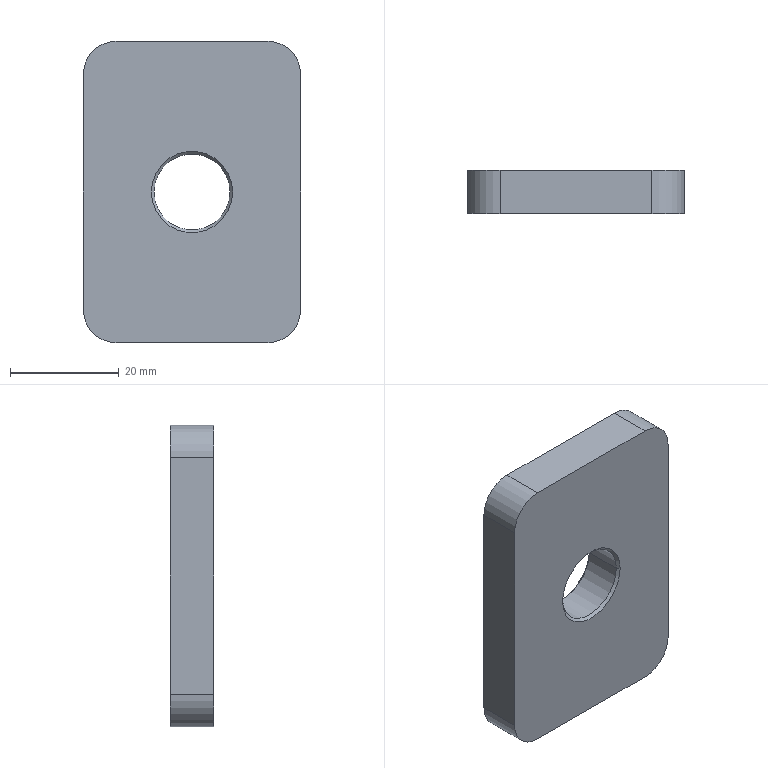Component | SolidWorks | 01-04RearWheelConnectionPlate-4 | 1 solid | 16 faces | box 40 x 8 x 55.5 mm | volume 16270 mm3 | cylinder 6 | plane 6 | cone 4 | commonest cylinder face diameters 12 x4 14 x2 | material Q235
STEP:
#1=CARTESIAN_POINT('',(-12.087,-0.01969,-13.848));
#2=VERTEX_POINT('',#1);
#3=CARTESIAN_POINT('',(-11.535,-0.01969,-13.848));
#4=VERTEX_POINT('',#3);
#5=CARTESIAN_POINT('',(-11.811,-0.01969,-13.848));
#6=DIRECTION('',(-0.,1.,-0.));
#7=DIRECTION('',(-1.,0.,0.));
#8=AXIS2_PLACEMENT_3D('',#5,#6,#7);
#9=CIRCLE('',#8,0.2756);
#10=EDGE_CURVE('',#2,#4,#9,.T.);
#11=ORIENTED_EDGE('',*,*,#10,.F.);
#12=CARTESIAN_POINT('',(-12.106,-0.,-13.848));
#13=VERTEX_POINT('',#12);
#14=CARTESIAN_POINT('',(-12.087,-0.01969,-13.848));
#15=DIRECTION('',(-0.7071,0.7071,0.));
#16=VECTOR('',#15,39.37);
#17=LINE('',#14,#16);
#18=EDGE_CURVE('',#2,#13,#17,.T.);
#19=ORIENTED_EDGE('',*,*,#18,.T.);
#20=CARTESIAN_POINT('',(-11.516,-0.,-13.848));
#21=VERTEX_POINT('',#20);
#22=CARTESIAN_POINT('',(-11.811,-0.,-13.848));
#23=DIRECTION('',(0.,-1.,0.));
#24=DIRECTION('',(-1.,-0.,0.));
#25=AXIS2_PLACEMENT_3D('',#22,#23,#24);
#26=CIRCLE('',#25,0.2953);
#27=EDGE_CURVE('',#21,#13,#26,.T.);
#28=ORIENTED_EDGE('',*,*,#27,.F.);
#29=CARTESIAN_POINT('',(-11.535,-0.01969,-13.848));
#30=DIRECTION('',(0.7071,0.7071,-0.));
#31=VECTOR('',#30,39.37);
#32=LINE('',#29,#31);
#33=EDGE_CURVE('',#4,#21,#32,.T.);
#34=ORIENTED_EDGE('',*,*,#33,.F.);
#35=EDGE_LOOP('',(#11,#19,#28,#34));
#36=FACE_OUTER_BOUND('',#35,.T.);
#37=CARTESIAN_POINT('',(-11.811,-0.01969,-13.848));
#38=DIRECTION('',(-0.,1.,-0.));
#39=DIRECTION('',(1.,0.,0.));
#40=AXIS2_PLACEMENT_3D('',#37,#38,#39);
#41=CONICAL_SURFACE('',#40,0.2756,0.7854);
#42=ADVANCED_FACE('',(#36),#41,.F.);
#43=CARTESIAN_POINT('',(-11.535,-0.2953,-13.848));
#44=VERTEX_POINT('',#43);
#45=CARTESIAN_POINT('',(-12.087,-0.2953,-13.848));
#46=VERTEX_POINT('',#45);
#47=CARTESIAN_POINT('',(-11.811,-0.2953,-13.848));
#48=DIRECTION('',(0.,-1.,0.));
#49=DIRECTION('',(-1.,0.,0.));
#50=AXIS2_PLACEMENT_3D('',#47,#48,#49);
#51=CIRCLE('',#50,0.2756);
#52=EDGE_CURVE('',#44,#46,#51,.T.);
#53=ORIENTED_EDGE('',*,*,#52,.F.);
#54=CARTESIAN_POINT('',(-11.516,-0.315,-13.848));
#55=VERTEX_POINT('',#54);
#56=CARTESIAN_POINT('',(-11.535,-0.2953,-13.848));
#57=DIRECTION('',(0.7071,-0.7071,-0.));
#58=VECTOR('',#57,39.37);
#59=LINE('',#56,#58);
#60=EDGE_CURVE('',#44,#55,#59,.T.);
#61=ORIENTED_EDGE('',*,*,#60,.T.);
#62=CARTESIAN_POINT('',(-12.106,-0.315,-13.848));
#63=VERTEX_POINT('',#62);
#64=CARTESIAN_POINT('',(-11.811,-0.315,-13.848));
#65=DIRECTION('',(-0.,1.,-0.));
#66=DIRECTION('',(-1.,0.,0.));
#67=AXIS2_PLACEMENT_3D('',#64,#65,#66);
#68=CIRCLE('',#67,0.2953);
#69=EDGE_CURVE('',#63,#55,#68,.T.);
#70=ORIENTED_EDGE('',*,*,#69,.F.);
#71=CARTESIAN_POINT('',(-12.087,-0.2953,-13.848));
#72=DIRECTION('',(-0.7071,-0.7071,0.));
#73=VECTOR('',#72,39.37);
#74=LINE('',#71,#73);
#75=EDGE_CURVE('',#46,#63,#74,.T.);
#76=ORIENTED_EDGE('',*,*,#75,.F.);
#77=EDGE_LOOP('',(#53,#61,#70,#76));
#78=FACE_OUTER_BOUND('',#77,.T.);
#79=CARTESIAN_POINT('',(-11.811,-0.2953,-13.848));
#80=DIRECTION('',(0.,-1.,0.));
#81=DIRECTION('',(-1.,0.,0.));
#82=AXIS2_PLACEMENT_3D('',#79,#80,#81);
#83=CONICAL_SURFACE('',#82,0.2756,0.7854);
#84=ADVANCED_FACE('',(#78),#83,.F.);
#85=ORIENTED_EDGE('',*,*,#52,.T.);
#86=CARTESIAN_POINT('',(-12.087,-0.,-13.848));
#87=DIRECTION('',(-0.,1.,-0.));
#88=VECTOR('',#87,39.37);
#89=LINE('',#86,#88);
#90=EDGE_CURVE('',#46,#2,#89,.T.);
#91=ORIENTED_EDGE('',*,*,#90,.T.);
#92=ORIENTED_EDGE('',*,*,#10,.T.);
#93=CARTESIAN_POINT('',(-11.535,-0.,-13.848));
#94=DIRECTION('',(-0.,1.,-0.));
#95=VECTOR('',#94,39.37);
#96=LINE('',#93,#95);
#97=EDGE_CURVE('',#44,#4,#96,.T.);
#98=ORIENTED_EDGE('',*,*,#97,.F.);
#99=EDGE_LOOP('',(#85,#91,#92,#98));
#100=FACE_OUTER_BOUND('',#99,.T.);
#101=CARTESIAN_POINT('',(-11.811,-0.,-13.848));
#102=DIRECTION('',(-0.,1.,-0.));
#103=DIRECTION('',(1.,0.,0.));
#104=AXIS2_PLACEMENT_3D('',#101,#102,#103);
#105=CYLINDRICAL_SURFACE('',#104,0.2756);
#106=ADVANCED_FACE('',(#100),#105,.F.);
#107=ORIENTED_EDGE('',*,*,#27,.T.);
#108=CARTESIAN_POINT('',(-11.811,-0.,-13.848));
#109=DIRECTION('',(0.,-1.,0.));
#110=DIRECTION('',(-1.,-0.,0.));
#111=AXIS2_PLACEMENT_3D('',#108,#109,#110);
#112=CIRCLE('',#111,0.2953);
#113=EDGE_CURVE('',#13,#21,#112,.T.);
#114=ORIENTED_EDGE('',*,*,#113,.T.);
#115=EDGE_LOOP('',(#107,#114));
#116=FACE_BOUND('',#115,.T.);
#117=CARTESIAN_POINT('',(-11.26,-0.,-14.941));
#118=VERTEX_POINT('',#117);
#119=CARTESIAN_POINT('',(-11.024,-0.,-14.705));
#120=VERTEX_POINT('',#119);
#121=CARTESIAN_POINT('',(-11.26,-0.,-14.705));
#122=DIRECTION('',(0.,-1.,0.));
#123=DIRECTION('',(-1.,-0.,0.));
#124=AXIS2_PLACEMENT_3D('',#121,#122,#123);
#125=CIRCLE('',#124,0.2362);
#126=EDGE_CURVE('',#118,#120,#125,.T.);
#127=ORIENTED_EDGE('',*,*,#126,.F.);
#128=CARTESIAN_POINT('',(-12.362,-0.,-14.941));
#129=VERTEX_POINT('',#128);
#130=CARTESIAN_POINT('',(-12.362,-0.,-14.941));
#131=DIRECTION('',(1.,0.,-0.));
#132=VECTOR('',#131,39.37);
#133=LINE('',#130,#132);
#134=EDGE_CURVE('',#129,#118,#133,.T.);
#135=ORIENTED_EDGE('',*,*,#134,.F.);
#136=CARTESIAN_POINT('',(-12.598,-0.,-14.705));
#137=VERTEX_POINT('',#136);
#138=CARTESIAN_POINT('',(-12.362,-0.,-14.705));
#139=DIRECTION('',(0.,-1.,0.));
#140=DIRECTION('',(1.,0.,0.));
#141=AXIS2_PLACEMENT_3D('',#138,#139,#140);
#142=CIRCLE('',#141,0.2362);
#143=EDGE_CURVE('',#137,#129,#142,.T.);
#144=ORIENTED_EDGE('',*,*,#143,.F.);
#145=CARTESIAN_POINT('',(-12.598,-0.,-12.992));
#146=VERTEX_POINT('',#145);
#147=CARTESIAN_POINT('',(-12.598,-0.,-14.705));
#148=DIRECTION('',(-0.,-0.,-1.));
#149=VECTOR('',#148,39.37);
#150=LINE('',#147,#149);
#151=EDGE_CURVE('',#146,#137,#150,.T.);
#152=ORIENTED_EDGE('',*,*,#151,.F.);
#153=CARTESIAN_POINT('',(-12.362,-0.,-12.756));
#154=VERTEX_POINT('',#153);
#155=CARTESIAN_POINT('',(-12.362,-0.,-12.992));
#156=DIRECTION('',(0.,-1.,0.));
#157=DIRECTION('',(1.,0.,0.));
#158=AXIS2_PLACEMENT_3D('',#155,#156,#157);
#159=CIRCLE('',#158,0.2362);
#160=EDGE_CURVE('',#154,#146,#159,.T.);
#161=ORIENTED_EDGE('',*,*,#160,.F.);
#162=CARTESIAN_POINT('',(-11.26,-0.,-12.756));
#163=VERTEX_POINT('',#162);
#164=CARTESIAN_POINT('',(-12.362,-0.,-12.756));
#165=DIRECTION('',(-1.,-0.,0.));
#166=VECTOR('',#165,39.37);
#167=LINE('',#164,#166);
#168=EDGE_CURVE('',#163,#154,#167,.T.);
#169=ORIENTED_EDGE('',*,*,#168,.F.);
#170=CARTESIAN_POINT('',(-11.024,-0.,-12.992));
#171=VERTEX_POINT('',#170);
#172=CARTESIAN_POINT('',(-11.26,-0.,-12.992));
#173=DIRECTION('',(0.,-1.,0.));
#174=DIRECTION('',(1.,0.,0.));
#175=AXIS2_PLACEMENT_3D('',#172,#173,#174);
#176=CIRCLE('',#175,0.2362);
#177=EDGE_CURVE('',#171,#163,#176,.T.);
#178=ORIENTED_EDGE('',*,*,#177,.F.);
#179=CARTESIAN_POINT('',(-11.024,-0.,-14.705));
#180=DIRECTION('',(0.,0.,1.));
#181=VECTOR('',#180,39.37);
#182=LINE('',#179,#181);
#183=EDGE_CURVE('',#120,#171,#182,.T.);
#184=ORIENTED_EDGE('',*,*,#183,.F.);
#185=EDGE_LOOP('',(#127,#135,#144,#152,#161,#169,#178,#184));
#186=FACE_OUTER_BOUND('',#185,.T.);
#187=CARTESIAN_POINT('',(-11.26,-0.,-14.705));
#188=DIRECTION('',(0.,-1.,0.));
#189=DIRECTION('',(-1.,-0.,0.));
#190=AXIS2_PLACEMENT_3D('',#187,#188,#189);
#191=PLANE('',#190);
#192=ADVANCED_FACE('',(#116,#186),#191,.F.);
#193=CARTESIAN_POINT('',(-11.26,-0.315,-14.941));
#194=VERTEX_POINT('',#193);
#195=CARTESIAN_POINT('',(-11.024,-0.315,-14.705));
#196=VERTEX_POINT('',#195);
#197=CARTESIAN_POINT('',(-11.26,-0.315,-14.705));
#198=DIRECTION('',(0.,-1.,0.));
#199=DIRECTION('',(-1.,0.,0.));
#200=AXIS2_PLACEMENT_3D('',#197,#198,#199);
#201=CIRCLE('',#200,0.2362);
#202=EDGE_CURVE('',#194,#196,#201,.T.);
#203=ORIENTED_EDGE('',*,*,#202,.F.);
#204=CARTESIAN_POINT('',(-11.26,-0.,-14.941));
#205=DIRECTION('',(0.,-1.,0.));
#206=VECTOR('',#205,39.37);
#207=LINE('',#204,#206);
#208=EDGE_CURVE('',#118,#194,#207,.T.);
#209=ORIENTED_EDGE('',*,*,#208,.F.);
#210=ORIENTED_EDGE('',*,*,#126,.T.);
#211=CARTESIAN_POINT('',(-11.024,-0.,-14.705));
#212=DIRECTION('',(0.,-1.,0.));
#213=VECTOR('',#212,39.37);
#214=LINE('',#211,#213);
#215=EDGE_CURVE('',#120,#196,#214,.T.);
#216=ORIENTED_EDGE('',*,*,#215,.T.);
#217=EDGE_LOOP('',(#203,#209,#210,#216));
#218=FACE_OUTER_BOUND('',#217,.T.);
#219=CARTESIAN_POINT('',(-11.26,-0.,-14.705));
#220=DIRECTION('',(0.,-1.,0.));
#221=DIRECTION('',(-1.,-0.,0.));
#222=AXIS2_PLACEMENT_3D('',#219,#220,#221);
#223=CYLINDRICAL_SURFACE('',#222,0.2362);
#224=ADVANCED_FACE('',(#218),#223,.T.);
#225=CARTESIAN_POINT('',(-12.362,-0.315,-14.941));
#226=VERTEX_POINT('',#225);
#227=CARTESIAN_POINT('',(-12.362,-0.315,-14.941));
#228=DIRECTION('',(1.,0.,-0.));
#229=VECTOR('',#228,39.37);
#230=LINE('',#227,#229);
#231=EDGE_CURVE('',#226,#194,#230,.T.);
#232=ORIENTED_EDGE('',*,*,#231,.F.);
#233=CARTESIAN_POINT('',(-12.362,-0.,-14.941));
#234=DIRECTION('',(0.,-1.,0.));
#235=VECTOR('',#234,39.37);
#236=LINE('',#233,#235);
#237=EDGE_CURVE('',#129,#226,#236,.T.);
#238=ORIENTED_EDGE('',*,*,#237,.F.);
#239=ORIENTED_EDGE('',*,*,#134,.T.);
#240=ORIENTED_EDGE('',*,*,#208,.T.);
#241=EDGE_LOOP('',(#232,#238,#239,#240));
#242=FACE_OUTER_BOUND('',#241,.T.);
#243=CARTESIAN_POINT('',(-12.362,-0.,-14.941));
#244=DIRECTION('',(-0.,-0.,-1.));
#245=DIRECTION('',(1.,0.,-0.));
#246=AXIS2_PLACEMENT_3D('',#243,#244,#245);
#247=PLANE('',#246);
#248=ADVANCED_FACE('',(#242),#247,.T.);
#249=CARTESIAN_POINT('',(-12.598,-0.315,-14.705));
#250=VERTEX_POINT('',#249);
#251=CARTESIAN_POINT('',(-12.362,-0.315,-14.705));
#252=DIRECTION('',(0.,-1.,0.));
#253=DIRECTION('',(1.,0.,0.));
#254=AXIS2_PLACEMENT_3D('',#251,#252,#253);
#255=CIRCLE('',#254,0.2362);
#256=EDGE_CURVE('',#250,#226,#255,.T.);
#257=ORIENTED_EDGE('',*,*,#256,.F.);
#258=CARTESIAN_POINT('',(-12.598,-0.,-14.705));
#259=DIRECTION('',(0.,-1.,0.));
#260=VECTOR('',#259,39.37);
#261=LINE('',#258,#260);
#262=EDGE_CURVE('',#137,#250,#261,.T.);
#263=ORIENTED_EDGE('',*,*,#262,.F.);
#264=ORIENTED_EDGE('',*,*,#143,.T.);
#265=ORIENTED_EDGE('',*,*,#237,.T.);
#266=EDGE_LOOP('',(#257,#263,#264,#265));
#267=FACE_OUTER_BOUND('',#266,.T.);
#268=CARTESIAN_POINT('',(-12.362,-0.,-14.705));
#269=DIRECTION('',(0.,-1.,0.));
#270=DIRECTION('',(-1.,-0.,0.));
#271=AXIS2_PLACEMENT_3D('',#268,#269,#270);
#272=CYLINDRICAL_SURFACE('',#271,0.2362);
#273=ADVANCED_FACE('',(#267),#272,.T.);
#274=CARTESIAN_POINT('',(-12.598,-0.315,-12.992));
#275=VERTEX_POINT('',#274);
#276=CARTESIAN_POINT('',(-12.598,-0.315,-14.705));
#277=DIRECTION('',(-0.,-0.,-1.));
#278=VECTOR('',#277,39.37);
#279=LINE('',#276,#278);
#280=EDGE_CURVE('',#275,#250,#279,.T.);
#281=ORIENTED_EDGE('',*,*,#280,.F.);
#282=CARTESIAN_POINT('',(-12.598,-0.,-12.992));
#283=DIRECTION('',(0.,-1.,0.));
#284=VECTOR('',#283,39.37);
#285=LINE('',#282,#284);
#286=EDGE_CURVE('',#146,#275,#285,.T.);
#287=ORIENTED_EDGE('',*,*,#286,.F.);
#288=ORIENTED_EDGE('',*,*,#151,.T.);
#289=ORIENTED_EDGE('',*,*,#262,.T.);
#290=EDGE_LOOP('',(#281,#287,#288,#289));
#291=FACE_OUTER_BOUND('',#290,.T.);
#292=CARTESIAN_POINT('',(-12.598,-0.,-14.705));
#293=DIRECTION('',(-1.,-0.,0.));
#294=DIRECTION('',(-0.,1.,-0.));
#295=AXIS2_PLACEMENT_3D('',#292,#293,#294);
#296=PLANE('',#295);
#297=ADVANCED_FACE('',(#291),#296,.T.);
#298=CARTESIAN_POINT('',(-12.362,-0.315,-12.756));
#299=VERTEX_POINT('',#298);
#300=CARTESIAN_POINT('',(-12.362,-0.315,-12.992));
#301=DIRECTION('',(0.,-1.,0.));
#302=DIRECTION('',(1.,0.,0.));
#303=AXIS2_PLACEMENT_3D('',#300,#301,#302);
#304=CIRCLE('',#303,0.2362);
#305=EDGE_CURVE('',#299,#275,#304,.T.);
#306=ORIENTED_EDGE('',*,*,#305,.F.);
#307=CARTESIAN_POINT('',(-12.362,-0.,-12.756));
#308=DIRECTION('',(0.,-1.,0.));
#309=VECTOR('',#308,39.37);
#310=LINE('',#307,#309);
#311=EDGE_CURVE('',#154,#299,#310,.T.);
#312=ORIENTED_EDGE('',*,*,#311,.F.);
#313=ORIENTED_EDGE('',*,*,#160,.T.);
#314=ORIENTED_EDGE('',*,*,#286,.T.);
#315=EDGE_LOOP('',(#306,#312,#313,#314));
#316=FACE_OUTER_BOUND('',#315,.T.);
#317=CARTESIAN_POINT('',(-12.362,-0.,-12.992));
#318=DIRECTION('',(0.,-1.,0.));
#319=DIRECTION('',(-1.,-0.,0.));
#320=AXIS2_PLACEMENT_3D('',#317,#318,#319);
#321=CYLINDRICAL_SURFACE('',#320,0.2362);
#322=ADVANCED_FACE('',(#316),#321,.T.);
#323=CARTESIAN_POINT('',(-11.26,-0.315,-12.756));
#324=VERTEX_POINT('',#323);
#325=CARTESIAN_POINT('',(-12.362,-0.315,-12.756));
#326=DIRECTION('',(-1.,-0.,0.));
#327=VECTOR('',#326,39.37);
#328=LINE('',#325,#327);
#329=EDGE_CURVE('',#324,#299,#328,.T.);
#330=ORIENTED_EDGE('',*,*,#329,.F.);
#331=CARTESIAN_POINT('',(-11.26,-0.,-12.756));
#332=DIRECTION('',(0.,-1.,0.));
#333=VECTOR('',#332,39.37);
#334=LINE('',#331,#333);
#335=EDGE_CURVE('',#163,#324,#334,.T.);
#336=ORIENTED_EDGE('',*,*,#335,.F.);
#337=ORIENTED_EDGE('',*,*,#168,.T.);
#338=ORIENTED_EDGE('',*,*,#311,.T.);
#339=EDGE_LOOP('',(#330,#336,#337,#338));
#340=FACE_OUTER_BOUND('',#339,.T.);
#341=CARTESIAN_POINT('',(-12.362,-0.,-12.756));
#342=DIRECTION('',(0.,0.,1.));
#343=DIRECTION('',(-1.,-0.,0.));
#344=AXIS2_PLACEMENT_3D('',#341,#342,#343);
#345=PLANE('',#344);
#346=ADVANCED_FACE('',(#340),#345,.T.);
#347=CARTESIAN_POINT('',(-11.024,-0.315,-12.992));
#348=VERTEX_POINT('',#347);
#349=CARTESIAN_POINT('',(-11.26,-0.315,-12.992));
#350=DIRECTION('',(0.,-1.,0.));
#351=DIRECTION('',(1.,0.,0.));
#352=AXIS2_PLACEMENT_3D('',#349,#350,#351);
#353=CIRCLE('',#352,0.2362);
#354=EDGE_CURVE('',#348,#324,#353,.T.);
#355=ORIENTED_EDGE('',*,*,#354,.F.);
#356=CARTESIAN_POINT('',(-11.024,-0.,-12.992));
#357=DIRECTION('',(0.,-1.,0.));
#358=VECTOR('',#357,39.37);
#359=LINE('',#356,#358);
#360=EDGE_CURVE('',#171,#348,#359,.T.);
#361=ORIENTED_EDGE('',*,*,#360,.F.);
#362=ORIENTED_EDGE('',*,*,#177,.T.);
#363=ORIENTED_EDGE('',*,*,#335,.T.);
#364=EDGE_LOOP('',(#355,#361,#362,#363));
#365=FACE_OUTER_BOUND('',#364,.T.);
#366=CARTESIAN_POINT('',(-11.26,-0.,-12.992));
#367=DIRECTION('',(0.,-1.,0.));
#368=DIRECTION('',(-1.,-0.,0.));
#369=AXIS2_PLACEMENT_3D('',#366,#367,#368);
#370=CYLINDRICAL_SURFACE('',#369,0.2362);
#371=ADVANCED_FACE('',(#365),#370,.T.);
#372=CARTESIAN_POINT('',(-11.024,-0.315,-14.705));
#373=DIRECTION('',(0.,0.,1.));
#374=VECTOR('',#373,39.37);
#375=LINE('',#372,#374);
#376=EDGE_CURVE('',#196,#348,#375,.T.);
#377=ORIENTED_EDGE('',*,*,#376,.F.);
#378=ORIENTED_EDGE('',*,*,#215,.F.);
#379=ORIENTED_EDGE('',*,*,#183,.T.);
#380=ORIENTED_EDGE('',*,*,#360,.T.);
#381=EDGE_LOOP('',(#377,#378,#379,#380));
#382=FACE_OUTER_BOUND('',#381,.T.);
#383=CARTESIAN_POINT('',(-11.024,-0.,-14.705));
#384=DIRECTION('',(1.,0.,-0.));
#385=DIRECTION('',(0.,0.,1.));
#386=AXIS2_PLACEMENT_3D('',#383,#384,#385);
#387=PLANE('',#386);
#388=ADVANCED_FACE('',(#382),#387,.T.);
#389=ORIENTED_EDGE('',*,*,#69,.T.);
#390=CARTESIAN_POINT('',(-11.811,-0.315,-13.848));
#391=DIRECTION('',(-0.,1.,-0.));
#392=DIRECTION('',(-1.,0.,0.));
#393=AXIS2_PLACEMENT_3D('',#390,#391,#392);
#394=CIRCLE('',#393,0.2953);
#395=EDGE_CURVE('',#55,#63,#394,.T.);
#396=ORIENTED_EDGE('',*,*,#395,.T.);
#397=EDGE_LOOP('',(#389,#396));
#398=FACE_BOUND('',#397,.T.);
#399=ORIENTED_EDGE('',*,*,#202,.T.);
#400=ORIENTED_EDGE('',*,*,#376,.T.);
#401=ORIENTED_EDGE('',*,*,#354,.T.);
#402=ORIENTED_EDGE('',*,*,#329,.T.);
#403=ORIENTED_EDGE('',*,*,#305,.T.);
#404=ORIENTED_EDGE('',*,*,#280,.T.);
#405=ORIENTED_EDGE('',*,*,#256,.T.);
#406=ORIENTED_EDGE('',*,*,#231,.T.);
#407=EDGE_LOOP('',(#399,#400,#401,#402,#403,#404,#405,#406));
#408=FACE_OUTER_BOUND('',#407,.T.);
#409=CARTESIAN_POINT('',(-11.26,-0.315,-14.705));
#410=DIRECTION('',(0.,-1.,0.));
#411=DIRECTION('',(-1.,-0.,0.));
#412=AXIS2_PLACEMENT_3D('',#409,#410,#411);
#413=PLANE('',#412);
#414=ADVANCED_FACE('',(#398,#408),#413,.T.);
#415=ORIENTED_EDGE('',*,*,#90,.F.);
#416=CARTESIAN_POINT('',(-11.811,-0.2953,-13.848));
#417=DIRECTION('',(0.,-1.,0.));
#418=DIRECTION('',(-1.,0.,0.));
#419=AXIS2_PLACEMENT_3D('',#416,#417,#418);
#420=CIRCLE('',#419,0.2756);
#421=EDGE_CURVE('',#46,#44,#420,.T.);
#422=ORIENTED_EDGE('',*,*,#421,.T.);
#423=ORIENTED_EDGE('',*,*,#97,.T.);
#424=CARTESIAN_POINT('',(-11.811,-0.01969,-13.848));
#425=DIRECTION('',(-0.,1.,-0.));
#426=DIRECTION('',(-1.,0.,0.));
#427=AXIS2_PLACEMENT_3D('',#424,#425,#426);
#428=CIRCLE('',#427,0.2756);
#429=EDGE_CURVE('',#4,#2,#428,.T.);
#430=ORIENTED_EDGE('',*,*,#429,.T.);
#431=EDGE_LOOP('',(#415,#422,#423,#430));
#432=FACE_OUTER_BOUND('',#431,.T.);
#433=CARTESIAN_POINT('',(-11.811,-0.,-13.848));
#434=DIRECTION('',(-0.,1.,-0.));
#435=DIRECTION('',(1.,0.,0.));
#436=AXIS2_PLACEMENT_3D('',#433,#434,#435);
#437=CYLINDRICAL_SURFACE('',#436,0.2756);
#438=ADVANCED_FACE('',(#432),#437,.F.);
#439=ORIENTED_EDGE('',*,*,#60,.F.);
#440=ORIENTED_EDGE('',*,*,#421,.F.);
#441=ORIENTED_EDGE('',*,*,#75,.T.);
#442=ORIENTED_EDGE('',*,*,#395,.F.);
#443=EDGE_LOOP('',(#439,#440,#441,#442));
#444=FACE_OUTER_BOUND('',#443,.T.);
#445=CARTESIAN_POINT('',(-11.811,-0.2953,-13.848));
#446=DIRECTION('',(0.,-1.,0.));
#447=DIRECTION('',(-1.,0.,0.));
#448=AXIS2_PLACEMENT_3D('',#445,#446,#447);
#449=CONICAL_SURFACE('',#448,0.2756,0.7854);
#450=ADVANCED_FACE('',(#444),#449,.F.);
#451=ORIENTED_EDGE('',*,*,#18,.F.);
#452=ORIENTED_EDGE('',*,*,#429,.F.);
#453=ORIENTED_EDGE('',*,*,#33,.T.);
#454=ORIENTED_EDGE('',*,*,#113,.F.);
#455=EDGE_LOOP('',(#451,#452,#453,#454));
#456=FACE_OUTER_BOUND('',#455,.T.);
#457=CARTESIAN_POINT('',(-11.811,-0.01969,-13.848));
#458=DIRECTION('',(-0.,1.,-0.));
#459=DIRECTION('',(1.,0.,0.));
#460=AXIS2_PLACEMENT_3D('',#457,#458,#459);
#461=CONICAL_SURFACE('',#460,0.2756,0.7854);
#462=ADVANCED_FACE('',(#456),#461,.F.);
#463=CLOSED_SHELL('',(#42,#84,#106,#192,#224,#248,#273,#297,#322,#346,#371,#388,#414,#438,#450,#462));
#464=MANIFOLD_SOLID_BREP('',#463);
#465=CARTESIAN_POINT('',(0.,0.,0.));
#466=DIRECTION('',(0.,0.,1.));
#467=DIRECTION('',(1.,0.,0.));
#468=AXIS2_PLACEMENT_3D('',#465,#466,#467);
#469=(LENGTH_UNIT()NAMED_UNIT(*)SI_UNIT($,.METRE.));
#470=LENGTH_MEASURE_WITH_UNIT(LENGTH_MEASURE(0.0254),#469);
#471=DIMENSIONAL_EXPONENTS(1.,0.,0.,0.,0.,0.,0.);
#472=(CONVERSION_BASED_UNIT('',#470)LENGTH_UNIT()NAMED_UNIT(#471));
#473=UNCERTAINTY_MEASURE_WITH_UNIT(LENGTH_MEASURE(0.00001),#472,'','');
#474=(NAMED_UNIT(*)PLANE_ANGLE_UNIT()SI_UNIT($,.RADIAN.));
#475=(NAMED_UNIT(*)SI_UNIT($,.STERADIAN.)SOLID_ANGLE_UNIT());
#476=(GEOMETRIC_REPRESENTATION_CONTEXT(3)GLOBAL_UNCERTAINTY_ASSIGNED_CONTEXT((#473))GLOBAL_UNIT_ASSIGNED_CONTEXT((#472,#474,#475))REPRESENTATION_CONTEXT('',''));
#477=ADVANCED_BREP_SHAPE_REPRESENTATION('',(#464,#468),#476);
#478=COLOUR_RGB('',0.7922,0.8196,0.9333);
#479=FILL_AREA_STYLE_COLOUR('',#478);
#480=FILL_AREA_STYLE('',(#479));
#481=SURFACE_STYLE_FILL_AREA(#480);
#482=SURFACE_SIDE_STYLE('',(#481));
#483=SURFACE_STYLE_USAGE(.BOTH.,#482);
#484=PRESENTATION_STYLE_ASSIGNMENT((#483));
#485=STYLED_ITEM('',(#484),#464);
#486=(LENGTH_UNIT()NAMED_UNIT(*)SI_UNIT($,.METRE.));
#487=LENGTH_MEASURE_WITH_UNIT(LENGTH_MEASURE(0.0254),#486);
#488=DIMENSIONAL_EXPONENTS(1.,0.,0.,0.,0.,0.,0.);
#489=(CONVERSION_BASED_UNIT('',#487)LENGTH_UNIT()NAMED_UNIT(#488));
#490=UNCERTAINTY_MEASURE_WITH_UNIT(LENGTH_MEASURE(0.00001),#489,'','');
#491=(NAMED_UNIT(*)PLANE_ANGLE_UNIT()SI_UNIT($,.RADIAN.));
#492=(NAMED_UNIT(*)SI_UNIT($,.STERADIAN.)SOLID_ANGLE_UNIT());
#493=(GEOMETRIC_REPRESENTATION_CONTEXT(3)GLOBAL_UNCERTAINTY_ASSIGNED_CONTEXT((#490))GLOBAL_UNIT_ASSIGNED_CONTEXT((#489,#491,#492))REPRESENTATION_CONTEXT('',''));
#494=MECHANICAL_DESIGN_GEOMETRIC_PRESENTATION_REPRESENTATION('',(#485),#493);
#495=PRESENTATION_LAYER_ASSIGNMENT('','',(#485));